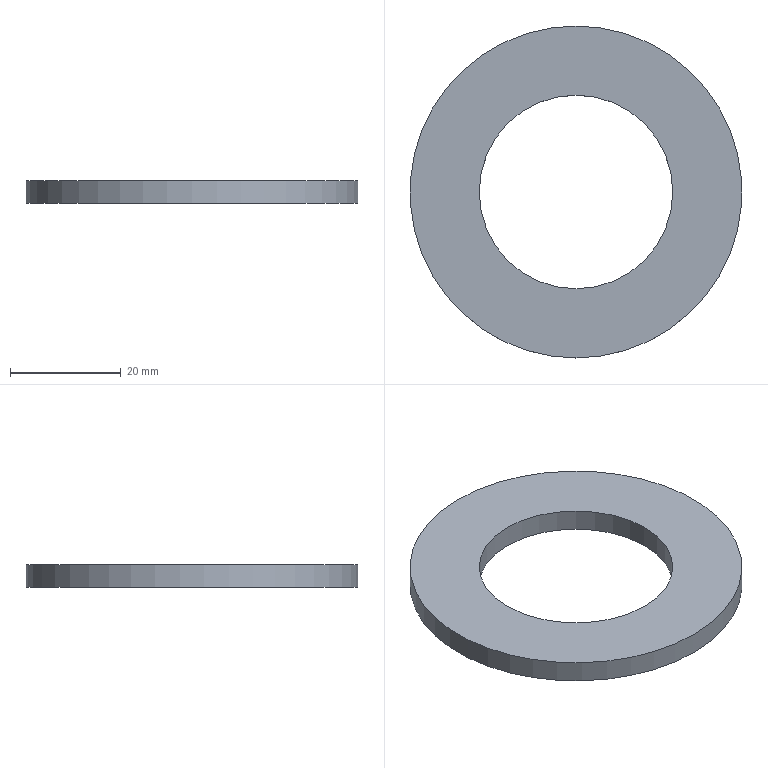Component | NX | CT-ZHOU5-DANGQUAN1 | 1 solid | 4 faces | box 60 x 60 x 4 mm | volume 7461 mm3 | cylinder 2 | plane 2 | commonest cylinder face diameters 60 x1 35 x1
STEP:
#1=CARTESIAN_POINT('',(0.,0.,0.));
#2=DIRECTION('',(0.,0.,1.));
#3=DIRECTION('',(1.,0.,0.));
#4=AXIS2_PLACEMENT_3D('',#1,#2,#3);
#5=CARTESIAN_POINT('',(0.,30.,-160.));
#6=VERTEX_POINT('',#5);
#7=CARTESIAN_POINT('',(0.,0.,-160.));
#8=DIRECTION('',(0.,0.,-1.));
#9=DIRECTION('',(-0.,1.,0.));
#10=AXIS2_PLACEMENT_3D('',#7,#8,#9);
#11=CIRCLE('',#10,30.);
#12=CARTESIAN_POINT('',(0.,0.,-160.));
#13=DIRECTION('',(0.,0.,1.));
#14=DIRECTION('',(1.,0.,0.));
#15=AXIS2_PLACEMENT_3D('',#12,#13,#14);
#16=CYLINDRICAL_SURFACE('',#15,30.);
#17=CARTESIAN_POINT('',(7.854,0.));
#18=DIRECTION('',(-1.,0.));
#19=VECTOR('',#18,1.);
#20=LINE('',#17,#19);
#21=(GEOMETRIC_REPRESENTATION_CONTEXT(2)PARAMETRIC_REPRESENTATION_CONTEXT()REPRESENTATION_CONTEXT('',''));
#22=DEFINITIONAL_REPRESENTATION('',(#20),#21);
#23=PCURVE('',#16,#22);
#24=CARTESIAN_POINT('',(0.,0.,-160.));
#25=DIRECTION('',(0.,0.,-1.));
#26=DIRECTION('',(-1.,0.,0.));
#27=AXIS2_PLACEMENT_3D('',#24,#25,#26);
#28=PLANE('',#27);
#29=CARTESIAN_POINT('',(0.,0.));
#30=DIRECTION('',(0.,1.));
#31=AXIS2_PLACEMENT_2D('',#29,#30);
#32=CIRCLE('',#31,30.);
#33=(GEOMETRIC_REPRESENTATION_CONTEXT(2)PARAMETRIC_REPRESENTATION_CONTEXT()REPRESENTATION_CONTEXT('',''));
#34=DEFINITIONAL_REPRESENTATION('',(#32),#33);
#35=PCURVE('',#28,#34);
#36=SURFACE_CURVE('',#11,(#23,#35),.PCURVE_S1.);
#37=EDGE_CURVE('',#6,#6,#36,.T.);
#38=ORIENTED_EDGE('',*,*,#37,.F.);
#39=CARTESIAN_POINT('',(0.,30.,-156.));
#40=VERTEX_POINT('',#39);
#41=CARTESIAN_POINT('',(0.,30.,-160.));
#42=CARTESIAN_POINT('',(0.,30.,-156.));
#43=B_SPLINE_CURVE_WITH_KNOTS('',1,(#41,#42),.UNSPECIFIED.,.F.,.F.,(2,2),(0.,4.),.PIECEWISE_BEZIER_KNOTS.);
#44=CARTESIAN_POINT('',(7.854,0.));
#45=DIRECTION('',(0.,1.));
#46=VECTOR('',#45,1.);
#47=LINE('',#44,#46);
#48=(GEOMETRIC_REPRESENTATION_CONTEXT(2)PARAMETRIC_REPRESENTATION_CONTEXT()REPRESENTATION_CONTEXT('',''));
#49=DEFINITIONAL_REPRESENTATION('',(#47),#48);
#50=PCURVE('',#16,#49);
#51=CARTESIAN_POINT('',(1.571,0.));
#52=DIRECTION('',(0.,1.));
#53=VECTOR('',#52,1.);
#54=LINE('',#51,#53);
#55=(GEOMETRIC_REPRESENTATION_CONTEXT(2)PARAMETRIC_REPRESENTATION_CONTEXT()REPRESENTATION_CONTEXT('',''));
#56=DEFINITIONAL_REPRESENTATION('',(#54),#55);
#57=PCURVE('',#16,#56);
#58=SEAM_CURVE('',#43,(#50,#57),.PCURVE_S1.);
#59=EDGE_CURVE('',#6,#40,#58,.T.);
#60=ORIENTED_EDGE('',*,*,#59,.T.);
#61=CARTESIAN_POINT('',(0.,0.,-156.));
#62=DIRECTION('',(0.,0.,-1.));
#63=DIRECTION('',(-0.,1.,0.));
#64=AXIS2_PLACEMENT_3D('',#61,#62,#63);
#65=CIRCLE('',#64,30.);
#66=CARTESIAN_POINT('',(7.854,4.));
#67=DIRECTION('',(-1.,0.));
#68=VECTOR('',#67,1.);
#69=LINE('',#66,#68);
#70=(GEOMETRIC_REPRESENTATION_CONTEXT(2)PARAMETRIC_REPRESENTATION_CONTEXT()REPRESENTATION_CONTEXT('',''));
#71=DEFINITIONAL_REPRESENTATION('',(#69),#70);
#72=PCURVE('',#16,#71);
#73=CARTESIAN_POINT('',(0.,0.,-156.));
#74=DIRECTION('',(0.,0.,-1.));
#75=DIRECTION('',(-1.,0.,0.));
#76=AXIS2_PLACEMENT_3D('',#73,#74,#75);
#77=PLANE('',#76);
#78=CARTESIAN_POINT('',(0.,0.));
#79=DIRECTION('',(0.,1.));
#80=AXIS2_PLACEMENT_2D('',#78,#79);
#81=CIRCLE('',#80,30.);
#82=(GEOMETRIC_REPRESENTATION_CONTEXT(2)PARAMETRIC_REPRESENTATION_CONTEXT()REPRESENTATION_CONTEXT('',''));
#83=DEFINITIONAL_REPRESENTATION('',(#81),#82);
#84=PCURVE('',#77,#83);
#85=SURFACE_CURVE('',#65,(#72,#84),.PCURVE_S1.);
#86=EDGE_CURVE('',#40,#40,#85,.T.);
#87=ORIENTED_EDGE('',*,*,#86,.T.);
#88=ORIENTED_EDGE('',*,*,#59,.F.);
#89=EDGE_LOOP('',(#38,#60,#87,#88));
#90=FACE_BOUND('',#89,.T.);
#91=ADVANCED_FACE('',(#90),#16,.T.);
#92=CARTESIAN_POINT('',(0.,17.5,-160.));
#93=VERTEX_POINT('',#92);
#94=CARTESIAN_POINT('',(0.,0.,-160.));
#95=DIRECTION('',(0.,0.,-1.));
#96=DIRECTION('',(-0.,1.,0.));
#97=AXIS2_PLACEMENT_3D('',#94,#95,#96);
#98=CIRCLE('',#97,17.5);
#99=CARTESIAN_POINT('',(0.,0.,-160.));
#100=DIRECTION('',(0.,0.,1.));
#101=DIRECTION('',(1.,0.,0.));
#102=AXIS2_PLACEMENT_3D('',#99,#100,#101);
#103=CYLINDRICAL_SURFACE('',#102,17.5);
#104=CARTESIAN_POINT('',(7.854,0.));
#105=DIRECTION('',(-1.,0.));
#106=VECTOR('',#105,1.);
#107=LINE('',#104,#106);
#108=(GEOMETRIC_REPRESENTATION_CONTEXT(2)PARAMETRIC_REPRESENTATION_CONTEXT()REPRESENTATION_CONTEXT('',''));
#109=DEFINITIONAL_REPRESENTATION('',(#107),#108);
#110=PCURVE('',#103,#109);
#111=CARTESIAN_POINT('',(0.,0.));
#112=DIRECTION('',(0.,1.));
#113=AXIS2_PLACEMENT_2D('',#111,#112);
#114=CIRCLE('',#113,17.5);
#115=(GEOMETRIC_REPRESENTATION_CONTEXT(2)PARAMETRIC_REPRESENTATION_CONTEXT()REPRESENTATION_CONTEXT('',''));
#116=DEFINITIONAL_REPRESENTATION('',(#114),#115);
#117=PCURVE('',#28,#116);
#118=SURFACE_CURVE('',#98,(#110,#117),.PCURVE_S1.);
#119=EDGE_CURVE('',#93,#93,#118,.T.);
#120=ORIENTED_EDGE('',*,*,#119,.F.);
#121=CARTESIAN_POINT('',(0.,17.5,-156.));
#122=VERTEX_POINT('',#121);
#123=CARTESIAN_POINT('',(0.,17.5,-160.));
#124=CARTESIAN_POINT('',(0.,17.5,-156.));
#125=B_SPLINE_CURVE_WITH_KNOTS('',1,(#123,#124),.UNSPECIFIED.,.F.,.F.,(2,2),(0.,4.),.PIECEWISE_BEZIER_KNOTS.);
#126=CARTESIAN_POINT('',(7.854,0.));
#127=DIRECTION('',(0.,1.));
#128=VECTOR('',#127,1.);
#129=LINE('',#126,#128);
#130=(GEOMETRIC_REPRESENTATION_CONTEXT(2)PARAMETRIC_REPRESENTATION_CONTEXT()REPRESENTATION_CONTEXT('',''));
#131=DEFINITIONAL_REPRESENTATION('',(#129),#130);
#132=PCURVE('',#103,#131);
#133=CARTESIAN_POINT('',(1.571,0.));
#134=DIRECTION('',(0.,1.));
#135=VECTOR('',#134,1.);
#136=LINE('',#133,#135);
#137=(GEOMETRIC_REPRESENTATION_CONTEXT(2)PARAMETRIC_REPRESENTATION_CONTEXT()REPRESENTATION_CONTEXT('',''));
#138=DEFINITIONAL_REPRESENTATION('',(#136),#137);
#139=PCURVE('',#103,#138);
#140=SEAM_CURVE('',#125,(#132,#139),.PCURVE_S1.);
#141=EDGE_CURVE('',#93,#122,#140,.T.);
#142=ORIENTED_EDGE('',*,*,#141,.T.);
#143=CARTESIAN_POINT('',(0.,0.,-156.));
#144=DIRECTION('',(0.,0.,-1.));
#145=DIRECTION('',(-0.,1.,0.));
#146=AXIS2_PLACEMENT_3D('',#143,#144,#145);
#147=CIRCLE('',#146,17.5);
#148=CARTESIAN_POINT('',(7.854,4.));
#149=DIRECTION('',(-1.,0.));
#150=VECTOR('',#149,1.);
#151=LINE('',#148,#150);
#152=(GEOMETRIC_REPRESENTATION_CONTEXT(2)PARAMETRIC_REPRESENTATION_CONTEXT()REPRESENTATION_CONTEXT('',''));
#153=DEFINITIONAL_REPRESENTATION('',(#151),#152);
#154=PCURVE('',#103,#153);
#155=CARTESIAN_POINT('',(0.,0.));
#156=DIRECTION('',(0.,1.));
#157=AXIS2_PLACEMENT_2D('',#155,#156);
#158=CIRCLE('',#157,17.5);
#159=(GEOMETRIC_REPRESENTATION_CONTEXT(2)PARAMETRIC_REPRESENTATION_CONTEXT()REPRESENTATION_CONTEXT('',''));
#160=DEFINITIONAL_REPRESENTATION('',(#158),#159);
#161=PCURVE('',#77,#160);
#162=SURFACE_CURVE('',#147,(#154,#161),.PCURVE_S1.);
#163=EDGE_CURVE('',#122,#122,#162,.T.);
#164=ORIENTED_EDGE('',*,*,#163,.T.);
#165=ORIENTED_EDGE('',*,*,#141,.F.);
#166=EDGE_LOOP('',(#120,#142,#164,#165));
#167=FACE_BOUND('',#166,.F.);
#168=ADVANCED_FACE('',(#167),#103,.F.);
#169=ORIENTED_EDGE('',*,*,#37,.T.);
#170=EDGE_LOOP('',(#169));
#171=FACE_BOUND('',#170,.T.);
#172=ORIENTED_EDGE('',*,*,#119,.F.);
#173=EDGE_LOOP('',(#172));
#174=FACE_BOUND('',#173,.T.);
#175=ADVANCED_FACE('',(#171,#174),#28,.T.);
#176=ORIENTED_EDGE('',*,*,#86,.F.);
#177=EDGE_LOOP('',(#176));
#178=FACE_BOUND('',#177,.T.);
#179=ORIENTED_EDGE('',*,*,#163,.T.);
#180=EDGE_LOOP('',(#179));
#181=FACE_BOUND('',#180,.T.);
#182=ADVANCED_FACE('',(#178,#181),#77,.F.);
#183=CLOSED_SHELL('',(#91,#168,#175,#182));
#184=MANIFOLD_SOLID_BREP('',#183);
#185=(LENGTH_UNIT()NAMED_UNIT(*)SI_UNIT(.MILLI.,.METRE.));
#186=UNCERTAINTY_MEASURE_WITH_UNIT(LENGTH_MEASURE(0.00001),#185,'','');
#187=(NAMED_UNIT(*)PLANE_ANGLE_UNIT()SI_UNIT($,.RADIAN.));
#188=(NAMED_UNIT(*)SI_UNIT($,.STERADIAN.)SOLID_ANGLE_UNIT());
#189=(GEOMETRIC_REPRESENTATION_CONTEXT(3)GLOBAL_UNCERTAINTY_ASSIGNED_CONTEXT((#186))GLOBAL_UNIT_ASSIGNED_CONTEXT((#185,#187,#188))REPRESENTATION_CONTEXT('',''));
#190=ADVANCED_BREP_SHAPE_REPRESENTATION('',(#4,#184),#189);